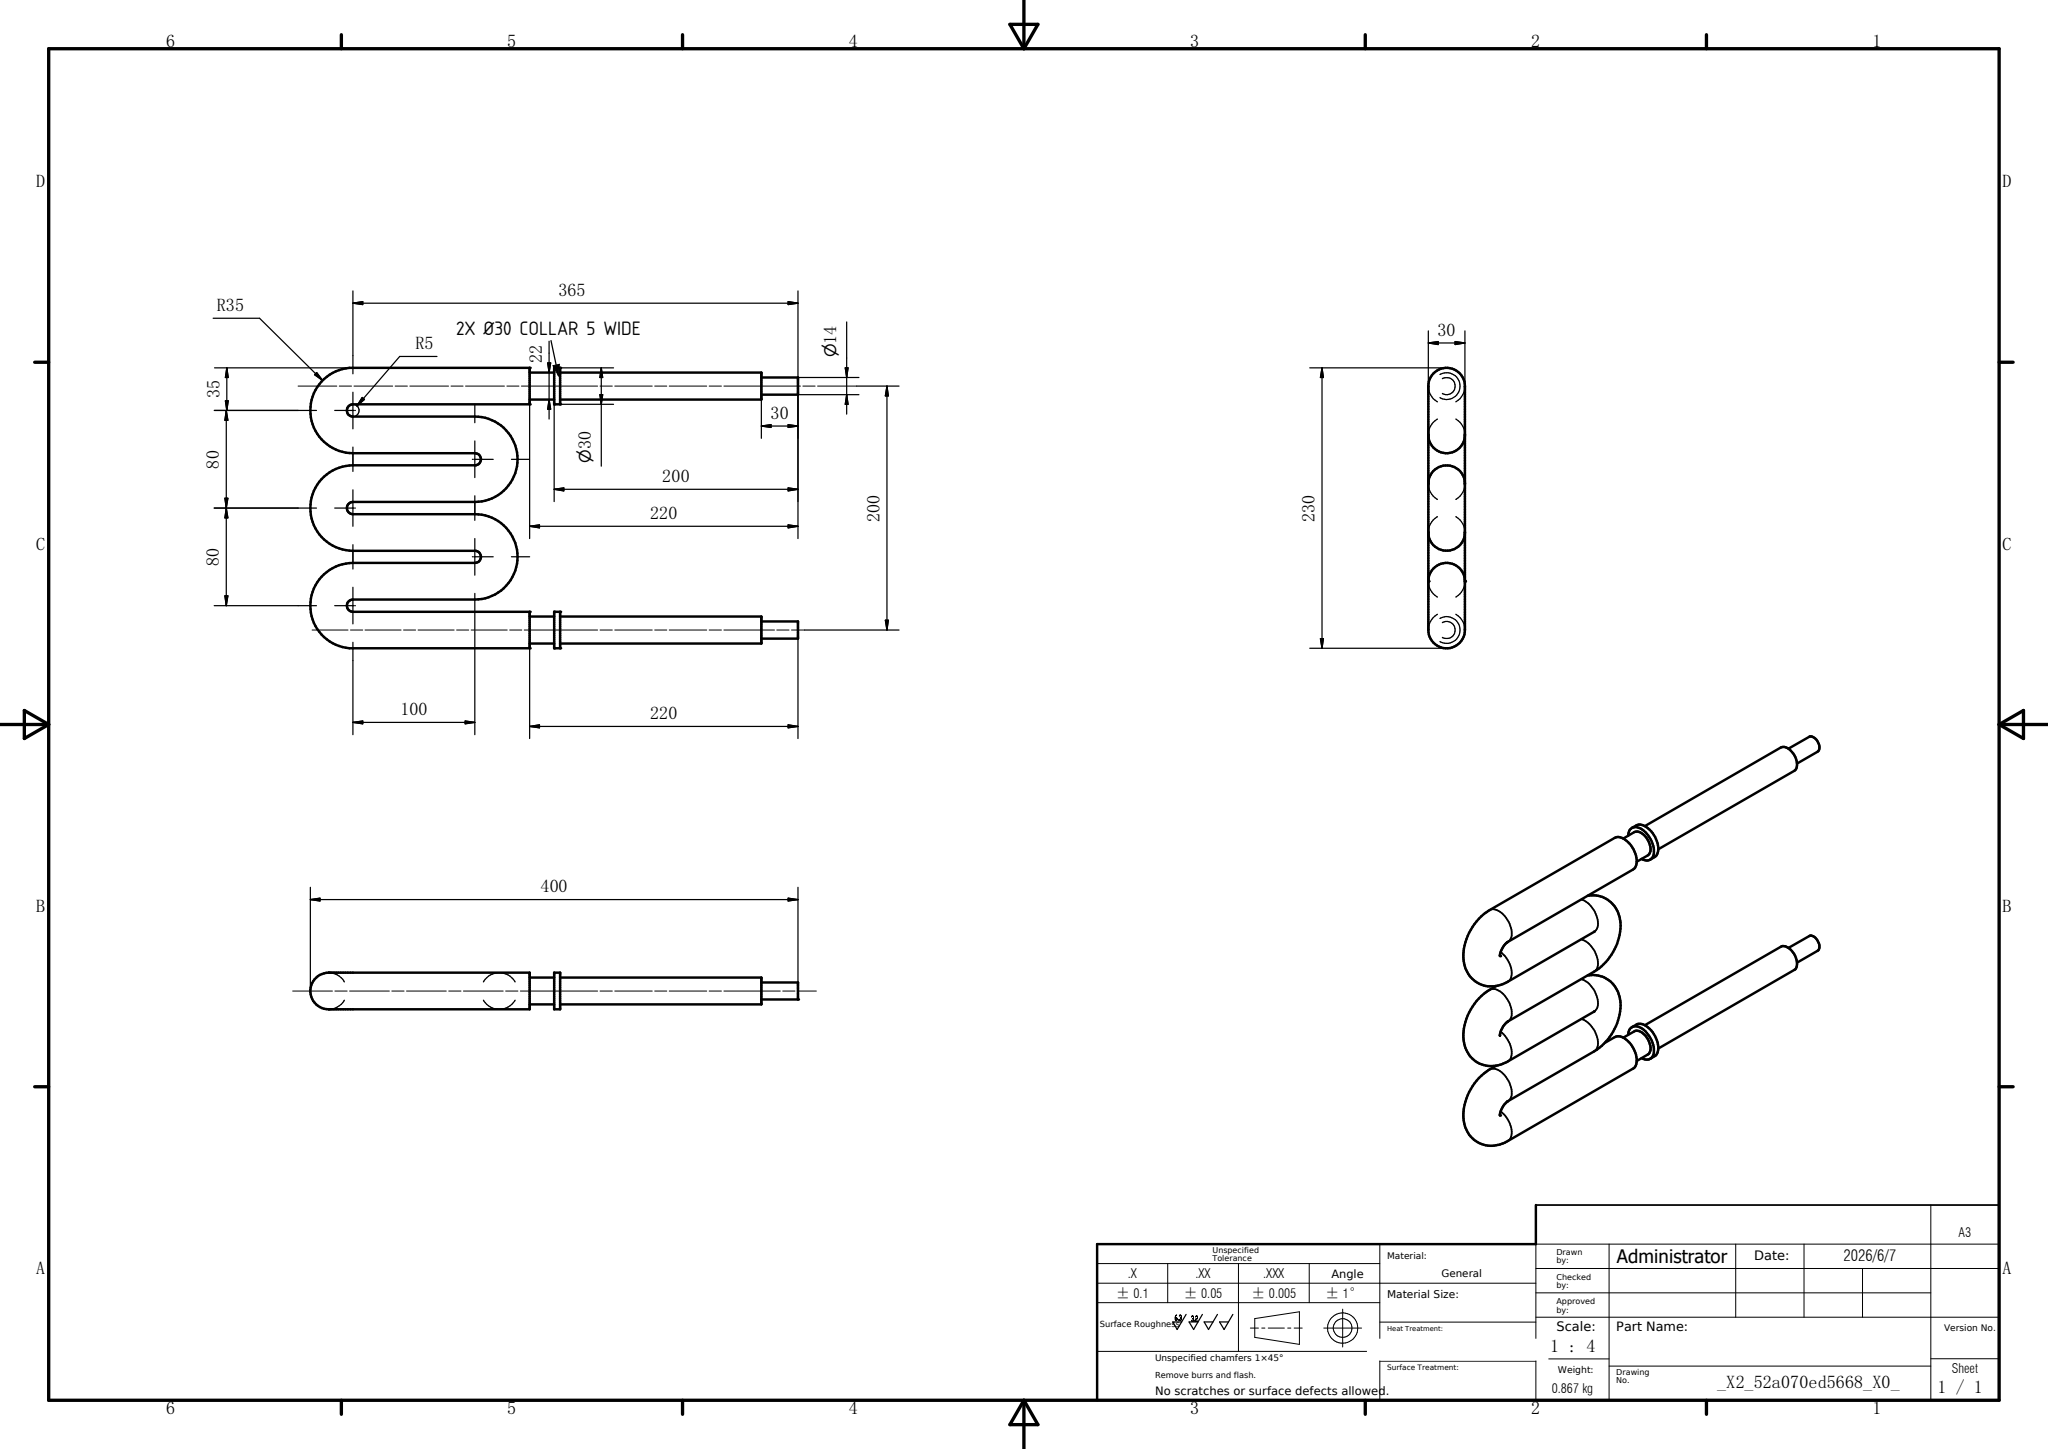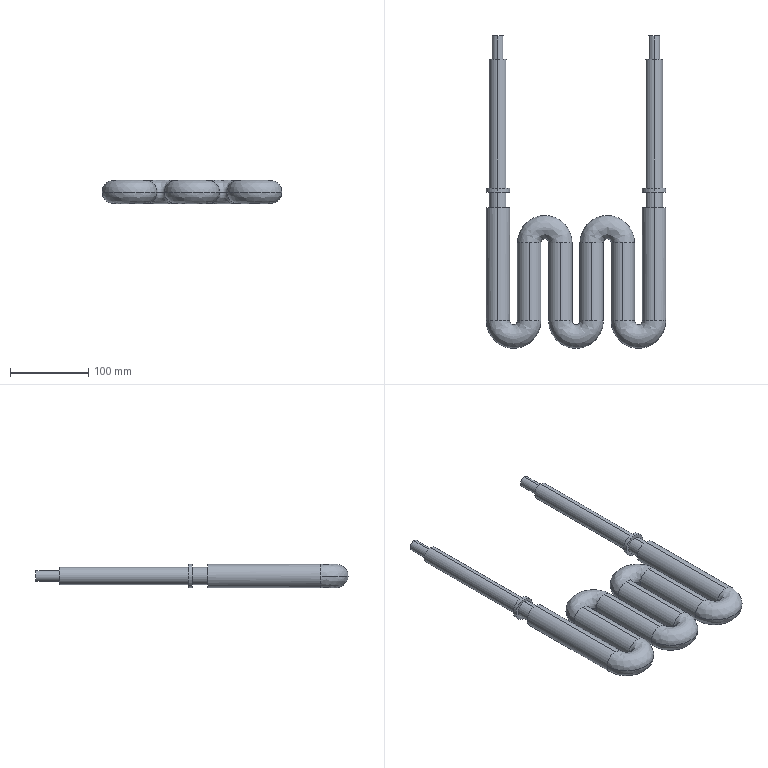Part | SolidWorks | mm | 1 solid | 48 faces | box 230 x 400 x 30 mm | volume 866752 mm3 | cylinder 28 | spline 10 | plane 10 | commonest cylinder face diameters 30 x16 22 x8 14 x4
Drawing notes:
Ø30 COLLAR 5 WIDE, BOTH SHAFTS; Ø22 165 LG FROM COLLAR TO Ø14 | from the solid: Ø30 cyl len 5.0 at y=235-240 (x=15 & 215); Ø22 cyl len 165 at y=240-405; Ø14 len 30 at y=405-435; 200 dim = 435-235